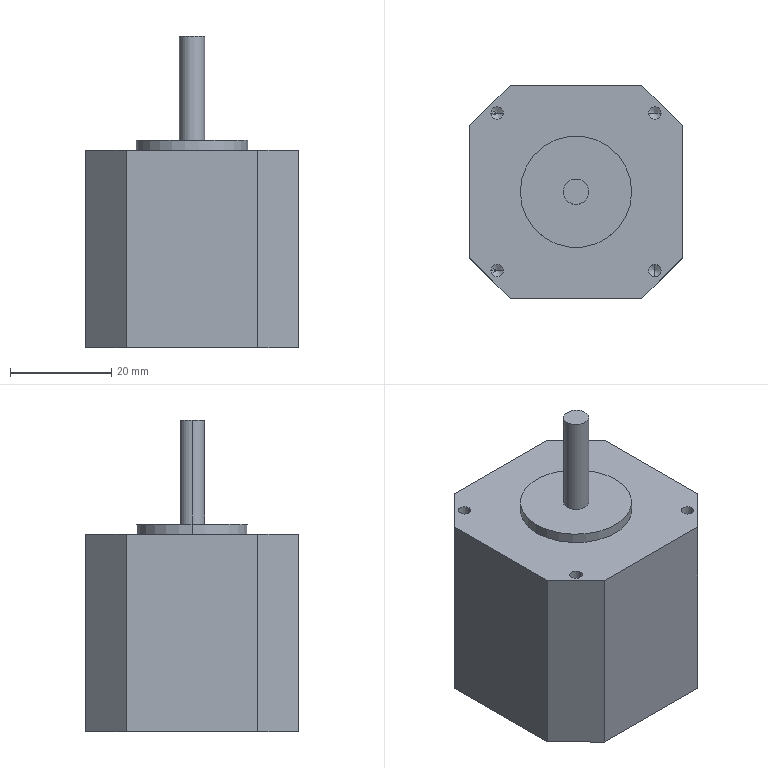Component | SolidWorks | 42StepperMotor-1 | 1 solid | 34 faces | box 42 x 42 x 61.5 mm | volume 64790 mm3 | cylinder 13 | plane 13 | cone 8 | commonest cylinder face diameters 2.5 x8 5 x3 22 x2
STEP:
#1=COLOUR_RGB('',0.7922,0.8196,0.9333);
#2=FILL_AREA_STYLE_COLOUR('',#1);
#3=FILL_AREA_STYLE('',(#2));
#4=SURFACE_STYLE_FILL_AREA(#3);
#5=SURFACE_SIDE_STYLE('',(#4));
#6=SURFACE_STYLE_USAGE(.BOTH.,#5);
#7=PRESENTATION_STYLE_ASSIGNMENT((#6));
#8=CARTESIAN_POINT('',(-0.4331,0.,0.07874));
#9=VERTEX_POINT('',#8);
#10=CARTESIAN_POINT('',(0.4331,0.,0.07874));
#11=VERTEX_POINT('',#10);
#12=CARTESIAN_POINT('',(-0.,0.,0.07874));
#13=DIRECTION('',(0.,0.,-1.));
#14=DIRECTION('',(-1.,0.,0.));
#15=AXIS2_PLACEMENT_3D('',#12,#13,#14);
#16=CIRCLE('',#15,0.4331);
#17=EDGE_CURVE('',#9,#11,#16,.T.);
#18=ORIENTED_EDGE('',*,*,#17,.T.);
#19=CARTESIAN_POINT('',(0.4331,0.,0.));
#20=VERTEX_POINT('',#19);
#21=CARTESIAN_POINT('',(0.4331,0.,0.07874));
#22=DIRECTION('',(0.,0.,-1.));
#23=VECTOR('',#22,39.37);
#24=LINE('',#21,#23);
#25=EDGE_CURVE('',#11,#20,#24,.T.);
#26=ORIENTED_EDGE('',*,*,#25,.T.);
#27=CARTESIAN_POINT('',(-0.4331,0.,0.));
#28=VERTEX_POINT('',#27);
#29=CARTESIAN_POINT('',(-0.,0.,0.));
#30=DIRECTION('',(0.,0.,1.));
#31=DIRECTION('',(-1.,0.,0.));
#32=AXIS2_PLACEMENT_3D('',#29,#30,#31);
#33=CIRCLE('',#32,0.4331);
#34=EDGE_CURVE('',#20,#28,#33,.T.);
#35=ORIENTED_EDGE('',*,*,#34,.T.);
#36=CARTESIAN_POINT('',(-0.4331,0.,0.07874));
#37=DIRECTION('',(0.,0.,-1.));
#38=VECTOR('',#37,39.37);
#39=LINE('',#36,#38);
#40=EDGE_CURVE('',#9,#28,#39,.T.);
#41=ORIENTED_EDGE('',*,*,#40,.F.);
#42=EDGE_LOOP('',(#18,#26,#35,#41));
#43=FACE_OUTER_BOUND('',#42,.T.);
#44=CARTESIAN_POINT('',(-0.,0.,0.07874));
#45=DIRECTION('',(0.,0.,-1.));
#46=DIRECTION('',(-1.,0.,0.));
#47=AXIS2_PLACEMENT_3D('',#44,#45,#46);
#48=CYLINDRICAL_SURFACE('',#47,0.4331);
#49=ADVANCED_FACE('',(#43),#48,.T.);
#50=CARTESIAN_POINT('',(-0.6617,0.6125,-0.3346));
#51=VERTEX_POINT('',#50);
#52=CARTESIAN_POINT('',(-0.5632,0.6125,-0.3346));
#53=VERTEX_POINT('',#52);
#54=CARTESIAN_POINT('',(-0.6125,0.6125,-0.3346));
#55=DIRECTION('',(0.,0.,1.));
#56=DIRECTION('',(1.,0.,0.));
#57=AXIS2_PLACEMENT_3D('',#54,#55,#56);
#58=CIRCLE('',#57,0.04921);
#59=EDGE_CURVE('',#51,#53,#58,.T.);
#60=ORIENTED_EDGE('',*,*,#59,.F.);
#61=CARTESIAN_POINT('',(-0.6617,0.6125,0.));
#62=VERTEX_POINT('',#61);
#63=CARTESIAN_POINT('',(-0.6617,0.6125,0.));
#64=DIRECTION('',(0.,0.,1.));
#65=VECTOR('',#64,39.37);
#66=LINE('',#63,#65);
#67=EDGE_CURVE('',#51,#62,#66,.T.);
#68=ORIENTED_EDGE('',*,*,#67,.T.);
#69=CARTESIAN_POINT('',(-0.5632,0.6125,0.));
#70=VERTEX_POINT('',#69);
#71=CARTESIAN_POINT('',(-0.6125,0.6125,0.));
#72=DIRECTION('',(0.,0.,1.));
#73=DIRECTION('',(1.,0.,0.));
#74=AXIS2_PLACEMENT_3D('',#71,#72,#73);
#75=CIRCLE('',#74,0.04921);
#76=EDGE_CURVE('',#62,#70,#75,.T.);
#77=ORIENTED_EDGE('',*,*,#76,.T.);
#78=CARTESIAN_POINT('',(-0.5632,0.6125,0.));
#79=DIRECTION('',(0.,0.,1.));
#80=VECTOR('',#79,39.37);
#81=LINE('',#78,#80);
#82=EDGE_CURVE('',#53,#70,#81,.T.);
#83=ORIENTED_EDGE('',*,*,#82,.F.);
#84=EDGE_LOOP('',(#60,#68,#77,#83));
#85=FACE_OUTER_BOUND('',#84,.T.);
#86=CARTESIAN_POINT('',(-0.6125,0.6125,0.));
#87=DIRECTION('',(0.,0.,1.));
#88=DIRECTION('',(1.,0.,0.));
#89=AXIS2_PLACEMENT_3D('',#86,#87,#88);
#90=CYLINDRICAL_SURFACE('',#89,0.04921);
#91=ADVANCED_FACE('',(#85),#90,.F.);
#92=CARTESIAN_POINT('',(0.5632,0.6125,-0.3346));
#93=VERTEX_POINT('',#92);
#94=CARTESIAN_POINT('',(0.6617,0.6125,-0.3346));
#95=VERTEX_POINT('',#94);
#96=CARTESIAN_POINT('',(0.6125,0.6125,-0.3346));
#97=DIRECTION('',(0.,0.,1.));
#98=DIRECTION('',(1.,0.,0.));
#99=AXIS2_PLACEMENT_3D('',#96,#97,#98);
#100=CIRCLE('',#99,0.04921);
#101=EDGE_CURVE('',#93,#95,#100,.T.);
#102=ORIENTED_EDGE('',*,*,#101,.F.);
#103=CARTESIAN_POINT('',(0.5632,0.6125,0.));
#104=VERTEX_POINT('',#103);
#105=CARTESIAN_POINT('',(0.5632,0.6125,0.));
#106=DIRECTION('',(0.,0.,1.));
#107=VECTOR('',#106,39.37);
#108=LINE('',#105,#107);
#109=EDGE_CURVE('',#93,#104,#108,.T.);
#110=ORIENTED_EDGE('',*,*,#109,.T.);
#111=CARTESIAN_POINT('',(0.6617,0.6125,0.));
#112=VERTEX_POINT('',#111);
#113=CARTESIAN_POINT('',(0.6125,0.6125,0.));
#114=DIRECTION('',(0.,0.,1.));
#115=DIRECTION('',(1.,0.,0.));
#116=AXIS2_PLACEMENT_3D('',#113,#114,#115);
#117=CIRCLE('',#116,0.04921);
#118=EDGE_CURVE('',#104,#112,#117,.T.);
#119=ORIENTED_EDGE('',*,*,#118,.T.);
#120=CARTESIAN_POINT('',(0.6617,0.6125,0.));
#121=DIRECTION('',(0.,0.,1.));
#122=VECTOR('',#121,39.37);
#123=LINE('',#120,#122);
#124=EDGE_CURVE('',#95,#112,#123,.T.);
#125=ORIENTED_EDGE('',*,*,#124,.F.);
#126=EDGE_LOOP('',(#102,#110,#119,#125));
#127=FACE_OUTER_BOUND('',#126,.T.);
#128=CARTESIAN_POINT('',(0.6125,0.6125,0.));
#129=DIRECTION('',(0.,0.,1.));
#130=DIRECTION('',(1.,0.,0.));
#131=AXIS2_PLACEMENT_3D('',#128,#129,#130);
#132=CYLINDRICAL_SURFACE('',#131,0.04921);
#133=ADVANCED_FACE('',(#127),#132,.F.);
#134=CARTESIAN_POINT('',(0.5632,-0.6125,-0.3346));
#135=VERTEX_POINT('',#134);
#136=CARTESIAN_POINT('',(0.6125,-0.6617,-0.3346));
#137=VERTEX_POINT('',#136);
#138=CARTESIAN_POINT('',(0.6125,-0.6125,-0.3346));
#139=DIRECTION('',(0.,0.,1.));
#140=DIRECTION('',(1.,0.,0.));
#141=AXIS2_PLACEMENT_3D('',#138,#139,#140);
#142=CIRCLE('',#141,0.04921);
#143=EDGE_CURVE('',#135,#137,#142,.T.);
#144=ORIENTED_EDGE('',*,*,#143,.F.);
#145=CARTESIAN_POINT('',(0.5632,-0.6125,0.));
#146=VERTEX_POINT('',#145);
#147=CARTESIAN_POINT('',(0.5632,-0.6125,0.));
#148=DIRECTION('',(0.,0.,1.));
#149=VECTOR('',#148,39.37);
#150=LINE('',#147,#149);
#151=EDGE_CURVE('',#135,#146,#150,.T.);
#152=ORIENTED_EDGE('',*,*,#151,.T.);
#153=CARTESIAN_POINT('',(0.6617,-0.6125,0.));
#154=VERTEX_POINT('',#153);
#155=CARTESIAN_POINT('',(0.6125,-0.6125,0.));
#156=DIRECTION('',(0.,0.,1.));
#157=DIRECTION('',(1.,0.,0.));
#158=AXIS2_PLACEMENT_3D('',#155,#156,#157);
#159=CIRCLE('',#158,0.04921);
#160=EDGE_CURVE('',#146,#154,#159,.T.);
#161=ORIENTED_EDGE('',*,*,#160,.T.);
#162=CARTESIAN_POINT('',(0.6617,-0.6125,-0.3346));
#163=VERTEX_POINT('',#162);
#164=CARTESIAN_POINT('',(0.6617,-0.6125,0.));
#165=DIRECTION('',(0.,0.,1.));
#166=VECTOR('',#165,39.37);
#167=LINE('',#164,#166);
#168=EDGE_CURVE('',#163,#154,#167,.T.);
#169=ORIENTED_EDGE('',*,*,#168,.F.);
#170=CARTESIAN_POINT('',(0.6125,-0.6125,-0.3346));
#171=DIRECTION('',(0.,0.,1.));
#172=DIRECTION('',(1.,0.,0.));
#173=AXIS2_PLACEMENT_3D('',#170,#171,#172);
#174=CIRCLE('',#173,0.04921);
#175=EDGE_CURVE('',#137,#163,#174,.T.);
#176=ORIENTED_EDGE('',*,*,#175,.F.);
#177=EDGE_LOOP('',(#144,#152,#161,#169,#176));
#178=FACE_OUTER_BOUND('',#177,.T.);
#179=CARTESIAN_POINT('',(0.6125,-0.6125,0.));
#180=DIRECTION('',(0.,0.,1.));
#181=DIRECTION('',(1.,0.,0.));
#182=AXIS2_PLACEMENT_3D('',#179,#180,#181);
#183=CYLINDRICAL_SURFACE('',#182,0.04921);
#184=ADVANCED_FACE('',(#178),#183,.F.);
#185=CARTESIAN_POINT('',(-0.6617,-0.6125,-0.3346));
#186=VERTEX_POINT('',#185);
#187=CARTESIAN_POINT('',(-0.5632,-0.6125,-0.3346));
#188=VERTEX_POINT('',#187);
#189=CARTESIAN_POINT('',(-0.6125,-0.6125,-0.3346));
#190=DIRECTION('',(0.,0.,1.));
#191=DIRECTION('',(1.,0.,0.));
#192=AXIS2_PLACEMENT_3D('',#189,#190,#191);
#193=CIRCLE('',#192,0.04921);
#194=EDGE_CURVE('',#186,#188,#193,.T.);
#195=ORIENTED_EDGE('',*,*,#194,.F.);
#196=CARTESIAN_POINT('',(-0.6617,-0.6125,0.));
#197=VERTEX_POINT('',#196);
#198=CARTESIAN_POINT('',(-0.6617,-0.6125,0.));
#199=DIRECTION('',(0.,0.,1.));
#200=VECTOR('',#199,39.37);
#201=LINE('',#198,#200);
#202=EDGE_CURVE('',#186,#197,#201,.T.);
#203=ORIENTED_EDGE('',*,*,#202,.T.);
#204=CARTESIAN_POINT('',(-0.5632,-0.6125,0.));
#205=VERTEX_POINT('',#204);
#206=CARTESIAN_POINT('',(-0.6125,-0.6125,0.));
#207=DIRECTION('',(0.,0.,1.));
#208=DIRECTION('',(1.,0.,0.));
#209=AXIS2_PLACEMENT_3D('',#206,#207,#208);
#210=CIRCLE('',#209,0.04921);
#211=EDGE_CURVE('',#197,#205,#210,.T.);
#212=ORIENTED_EDGE('',*,*,#211,.T.);
#213=CARTESIAN_POINT('',(-0.5632,-0.6125,0.));
#214=DIRECTION('',(0.,0.,1.));
#215=VECTOR('',#214,39.37);
#216=LINE('',#213,#215);
#217=EDGE_CURVE('',#188,#205,#216,.T.);
#218=ORIENTED_EDGE('',*,*,#217,.F.);
#219=EDGE_LOOP('',(#195,#203,#212,#218));
#220=FACE_OUTER_BOUND('',#219,.T.);
#221=CARTESIAN_POINT('',(-0.6125,-0.6125,0.));
#222=DIRECTION('',(0.,0.,1.));
#223=DIRECTION('',(1.,0.,0.));
#224=AXIS2_PLACEMENT_3D('',#221,#222,#223);
#225=CYLINDRICAL_SURFACE('',#224,0.04921);
#226=ADVANCED_FACE('',(#220),#225,.F.);
#227=CARTESIAN_POINT('',(-0.6125,0.6125,-0.3642));
#228=VERTEX_POINT('',#227);
#229=CARTESIAN_POINT('',(-0.5632,0.6125,-0.3346));
#230=DIRECTION('',(0.8572,0.,0.515));
#231=VECTOR('',#230,39.37);
#232=LINE('',#229,#231);
#233=EDGE_CURVE('',#228,#53,#232,.T.);
#234=ORIENTED_EDGE('',*,*,#233,.F.);
#235=CARTESIAN_POINT('',(-0.6617,0.6125,-0.3346));
#236=DIRECTION('',(-0.8572,0.,0.515));
#237=VECTOR('',#236,39.37);
#238=LINE('',#235,#237);
#239=EDGE_CURVE('',#228,#51,#238,.T.);
#240=ORIENTED_EDGE('',*,*,#239,.T.);
#241=ORIENTED_EDGE('',*,*,#59,.T.);
#242=EDGE_LOOP('',(#234,#240,#241));
#243=FACE_OUTER_BOUND('',#242,.T.);
#244=CARTESIAN_POINT('',(-0.6125,0.6125,-0.3346));
#245=DIRECTION('',(0.,0.,1.));
#246=DIRECTION('',(1.,0.,0.));
#247=AXIS2_PLACEMENT_3D('',#244,#245,#246);
#248=CONICAL_SURFACE('',#247,0.04921,1.03);
#249=ADVANCED_FACE('',(#243),#248,.F.);
#250=CARTESIAN_POINT('',(0.6125,0.6125,-0.3642));
#251=VERTEX_POINT('',#250);
#252=CARTESIAN_POINT('',(0.6617,0.6125,-0.3346));
#253=DIRECTION('',(0.8572,0.,0.515));
#254=VECTOR('',#253,39.37);
#255=LINE('',#252,#254);
#256=EDGE_CURVE('',#251,#95,#255,.T.);
#257=ORIENTED_EDGE('',*,*,#256,.F.);
#258=CARTESIAN_POINT('',(0.5632,0.6125,-0.3346));
#259=DIRECTION('',(-0.8572,0.,0.515));
#260=VECTOR('',#259,39.37);
#261=LINE('',#258,#260);
#262=EDGE_CURVE('',#251,#93,#261,.T.);
#263=ORIENTED_EDGE('',*,*,#262,.T.);
#264=ORIENTED_EDGE('',*,*,#101,.T.);
#265=EDGE_LOOP('',(#257,#263,#264));
#266=FACE_OUTER_BOUND('',#265,.T.);
#267=CARTESIAN_POINT('',(0.6125,0.6125,-0.3346));
#268=DIRECTION('',(0.,0.,1.));
#269=DIRECTION('',(1.,0.,0.));
#270=AXIS2_PLACEMENT_3D('',#267,#268,#269);
#271=CONICAL_SURFACE('',#270,0.04921,1.03);
#272=ADVANCED_FACE('',(#266),#271,.F.);
#273=CARTESIAN_POINT('',(0.6125,-0.6125,-0.3642));
#274=VERTEX_POINT('',#273);
#275=CARTESIAN_POINT('',(0.6125,-0.6617,-0.3346));
#276=DIRECTION('',(0.,-0.8572,0.515));
#277=VECTOR('',#276,39.37);
#278=LINE('',#275,#277);
#279=EDGE_CURVE('',#274,#137,#278,.T.);
#280=ORIENTED_EDGE('',*,*,#279,.F.);
#281=CARTESIAN_POINT('',(0.6125,-0.5632,-0.3346));
#282=VERTEX_POINT('',#281);
#283=CARTESIAN_POINT('',(0.6125,-0.5632,-0.3346));
#284=DIRECTION('',(0.,0.8572,0.515));
#285=VECTOR('',#284,39.37);
#286=LINE('',#283,#285);
#287=EDGE_CURVE('',#274,#282,#286,.T.);
#288=ORIENTED_EDGE('',*,*,#287,.T.);
#289=CARTESIAN_POINT('',(0.6125,-0.6125,-0.3346));
#290=DIRECTION('',(0.,0.,1.));
#291=DIRECTION('',(1.,0.,0.));
#292=AXIS2_PLACEMENT_3D('',#289,#290,#291);
#293=CIRCLE('',#292,0.04921);
#294=EDGE_CURVE('',#282,#135,#293,.T.);
#295=ORIENTED_EDGE('',*,*,#294,.T.);
#296=ORIENTED_EDGE('',*,*,#143,.T.);
#297=EDGE_LOOP('',(#280,#288,#295,#296));
#298=FACE_OUTER_BOUND('',#297,.T.);
#299=CARTESIAN_POINT('',(0.6125,-0.6125,-0.3346));
#300=DIRECTION('',(0.,0.,1.));
#301=DIRECTION('',(0.,-1.,0.));
#302=AXIS2_PLACEMENT_3D('',#299,#300,#301);
#303=CONICAL_SURFACE('',#302,0.04921,1.03);
#304=ADVANCED_FACE('',(#298),#303,.F.);
#305=CARTESIAN_POINT('',(-0.6125,-0.6125,-0.3642));
#306=VERTEX_POINT('',#305);
#307=CARTESIAN_POINT('',(-0.5632,-0.6125,-0.3346));
#308=DIRECTION('',(0.8572,0.,0.515));
#309=VECTOR('',#308,39.37);
#310=LINE('',#307,#309);
#311=EDGE_CURVE('',#306,#188,#310,.T.);
#312=ORIENTED_EDGE('',*,*,#311,.F.);
#313=CARTESIAN_POINT('',(-0.6617,-0.6125,-0.3346));
#314=DIRECTION('',(-0.8572,0.,0.515));
#315=VECTOR('',#314,39.37);
#316=LINE('',#313,#315);
#317=EDGE_CURVE('',#306,#186,#316,.T.);
#318=ORIENTED_EDGE('',*,*,#317,.T.);
#319=ORIENTED_EDGE('',*,*,#194,.T.);
#320=EDGE_LOOP('',(#312,#318,#319));
#321=FACE_OUTER_BOUND('',#320,.T.);
#322=CARTESIAN_POINT('',(-0.6125,-0.6125,-0.3346));
#323=DIRECTION('',(0.,0.,1.));
#324=DIRECTION('',(1.,0.,0.));
#325=AXIS2_PLACEMENT_3D('',#322,#323,#324);
#326=CONICAL_SURFACE('',#325,0.04921,1.03);
#327=ADVANCED_FACE('',(#321),#326,.F.);
#328=CARTESIAN_POINT('',(0.03857,0.09055,0.8858));
#329=VERTEX_POINT('',#328);
#330=CARTESIAN_POINT('',(0.09843,0.,0.8858));
#331=VERTEX_POINT('',#330);
#332=CARTESIAN_POINT('',(-0.,0.,0.8858));
#333=DIRECTION('',(0.,0.,-1.));
#334=DIRECTION('',(-1.,0.,0.));
#335=AXIS2_PLACEMENT_3D('',#332,#333,#334);
#336=CIRCLE('',#335,0.09843);
#337=EDGE_CURVE('',#329,#331,#336,.T.);
#338=ORIENTED_EDGE('',*,*,#337,.T.);
#339=CARTESIAN_POINT('',(0.09843,0.,0.07874));
#340=VERTEX_POINT('',#339);
#341=CARTESIAN_POINT('',(0.09843,0.,0.8858));
#342=DIRECTION('',(0.,0.,-1.));
#343=VECTOR('',#342,39.37);
#344=LINE('',#341,#343);
#345=EDGE_CURVE('',#331,#340,#344,.T.);
#346=ORIENTED_EDGE('',*,*,#345,.T.);
#347=CARTESIAN_POINT('',(0.03857,0.09055,0.07874));
#348=VERTEX_POINT('',#347);
#349=CARTESIAN_POINT('',(-0.,0.,0.07874));
#350=DIRECTION('',(0.,0.,-1.));
#351=DIRECTION('',(-1.,0.,0.));
#352=AXIS2_PLACEMENT_3D('',#349,#350,#351);
#353=CIRCLE('',#352,0.09843);
#354=EDGE_CURVE('',#348,#340,#353,.T.);
#355=ORIENTED_EDGE('',*,*,#354,.F.);
#356=CARTESIAN_POINT('',(0.03857,0.09055,0.8858));
#357=DIRECTION('',(0.,0.,1.));
#358=VECTOR('',#357,39.37);
#359=LINE('',#356,#358);
#360=EDGE_CURVE('',#348,#329,#359,.T.);
#361=ORIENTED_EDGE('',*,*,#360,.T.);
#362=EDGE_LOOP('',(#338,#346,#355,#361));
#363=FACE_OUTER_BOUND('',#362,.T.);
#364=CARTESIAN_POINT('',(-0.,0.,0.8858));
#365=DIRECTION('',(0.,0.,-1.));
#366=DIRECTION('',(-1.,0.,0.));
#367=AXIS2_PLACEMENT_3D('',#364,#365,#366);
#368=CYLINDRICAL_SURFACE('',#367,0.09843);
#369=ADVANCED_FACE('',(#363),#368,.T.);
#370=ORIENTED_EDGE('',*,*,#345,.F.);
#371=CARTESIAN_POINT('',(-0.09843,0.,0.8858));
#372=VERTEX_POINT('',#371);
#373=CARTESIAN_POINT('',(-0.,0.,0.8858));
#374=DIRECTION('',(0.,0.,-1.));
#375=DIRECTION('',(-1.,0.,0.));
#376=AXIS2_PLACEMENT_3D('',#373,#374,#375);
#377=CIRCLE('',#376,0.09843);
#378=EDGE_CURVE('',#331,#372,#377,.T.);
#379=ORIENTED_EDGE('',*,*,#378,.T.);
#380=CARTESIAN_POINT('',(-0.09843,0.,0.07874));
#381=VERTEX_POINT('',#380);
#382=CARTESIAN_POINT('',(-0.09843,0.,0.8858));
#383=DIRECTION('',(0.,0.,-1.));
#384=VECTOR('',#383,39.37);
#385=LINE('',#382,#384);
#386=EDGE_CURVE('',#372,#381,#385,.T.);
#387=ORIENTED_EDGE('',*,*,#386,.T.);
#388=CARTESIAN_POINT('',(-0.,0.,0.07874));
#389=DIRECTION('',(0.,0.,-1.));
#390=DIRECTION('',(-1.,0.,0.));
#391=AXIS2_PLACEMENT_3D('',#388,#389,#390);
#392=CIRCLE('',#391,0.09843);
#393=EDGE_CURVE('',#340,#381,#392,.T.);
#394=ORIENTED_EDGE('',*,*,#393,.F.);
#395=EDGE_LOOP('',(#370,#379,#387,#394));
#396=FACE_OUTER_BOUND('',#395,.T.);
#397=CARTESIAN_POINT('',(-0.,0.,0.8858));
#398=DIRECTION('',(0.,0.,-1.));
#399=DIRECTION('',(-1.,0.,0.));
#400=AXIS2_PLACEMENT_3D('',#397,#398,#399);
#401=CYLINDRICAL_SURFACE('',#400,0.09843);
#402=ADVANCED_FACE('',(#396),#401,.T.);
#403=CARTESIAN_POINT('',(-0.5118,0.8268,-1.535));
#404=VERTEX_POINT('',#403);
#405=CARTESIAN_POINT('',(0.5118,0.8268,-1.535));
#406=VERTEX_POINT('',#405);
#407=CARTESIAN_POINT('',(-0.,0.8268,-1.535));
#408=DIRECTION('',(1.,0.,0.));
#409=VECTOR('',#408,39.37);
#410=LINE('',#407,#409);
#411=EDGE_CURVE('',#404,#406,#410,.T.);
#412=ORIENTED_EDGE('',*,*,#411,.T.);
#413=CARTESIAN_POINT('',(0.8268,0.5118,-1.535));
#414=VERTEX_POINT('',#413);
#415=CARTESIAN_POINT('',(0.5118,0.8268,-1.535));
#416=DIRECTION('',(0.7071,-0.7071,0.));
#417=VECTOR('',#416,39.37);
#418=LINE('',#415,#417);
#419=EDGE_CURVE('',#406,#414,#418,.T.);
#420=ORIENTED_EDGE('',*,*,#419,.T.);
#421=CARTESIAN_POINT('',(0.8268,-0.5118,-1.535));
#422=VERTEX_POINT('',#421);
#423=CARTESIAN_POINT('',(0.8268,0.,-1.535));
#424=DIRECTION('',(0.,-1.,0.));
#425=VECTOR('',#424,39.37);
#426=LINE('',#423,#425);
#427=EDGE_CURVE('',#414,#422,#426,.T.);
#428=ORIENTED_EDGE('',*,*,#427,.T.);
#429=CARTESIAN_POINT('',(0.5118,-0.8268,-1.535));
#430=VERTEX_POINT('',#429);
#431=CARTESIAN_POINT('',(0.8268,-0.5118,-1.535));
#432=DIRECTION('',(-0.7071,-0.7071,0.));
#433=VECTOR('',#432,39.37);
#434=LINE('',#431,#433);
#435=EDGE_CURVE('',#422,#430,#434,.T.);
#436=ORIENTED_EDGE('',*,*,#435,.T.);
#437=CARTESIAN_POINT('',(-0.5118,-0.8268,-1.535));
#438=VERTEX_POINT('',#437);
#439=CARTESIAN_POINT('',(-0.,-0.8268,-1.535));
#440=DIRECTION('',(-1.,0.,0.));
#441=VECTOR('',#440,39.37);
#442=LINE('',#439,#441);
#443=EDGE_CURVE('',#430,#438,#442,.T.);
#444=ORIENTED_EDGE('',*,*,#443,.T.);
#445=CARTESIAN_POINT('',(-0.8268,-0.5118,-1.535));
#446=VERTEX_POINT('',#445);
#447=CARTESIAN_POINT('',(-0.5118,-0.8268,-1.535));
#448=DIRECTION('',(-0.7071,0.7071,0.));
#449=VECTOR('',#448,39.37);
#450=LINE('',#447,#449);
#451=EDGE_CURVE('',#438,#446,#450,.T.);
#452=ORIENTED_EDGE('',*,*,#451,.T.);
#453=CARTESIAN_POINT('',(-0.8268,0.5118,-1.535));
#454=VERTEX_POINT('',#453);
#455=CARTESIAN_POINT('',(-0.8268,0.,-1.535));
#456=DIRECTION('',(0.,1.,0.));
#457=VECTOR('',#456,39.37);
#458=LINE('',#455,#457);
#459=EDGE_CURVE('',#446,#454,#458,.T.);
#460=ORIENTED_EDGE('',*,*,#459,.T.);
#461=CARTESIAN_POINT('',(-0.8268,0.5118,-1.535));
#462=DIRECTION('',(0.7071,0.7071,0.));
#463=VECTOR('',#462,39.37);
#464=LINE('',#461,#463);
#465=EDGE_CURVE('',#454,#404,#464,.T.);
#466=ORIENTED_EDGE('',*,*,#465,.T.);
#467=EDGE_LOOP('',(#412,#420,#428,#436,#444,#452,#460,#466));
#468=FACE_OUTER_BOUND('',#467,.T.);
#469=CARTESIAN_POINT('',(-0.,0.,-1.535));
#470=DIRECTION('',(0.,0.,-1.));
#471=DIRECTION('',(-1.,0.,0.));
#472=AXIS2_PLACEMENT_3D('',#469,#470,#471);
#473=PLANE('',#472);
#474=ADVANCED_FACE('',(#468),#473,.T.);
#475=CARTESIAN_POINT('',(0.8268,0.5118,0.));
#476=VERTEX_POINT('',#475);
#477=CARTESIAN_POINT('',(0.8268,0.5118,0.));
#478=DIRECTION('',(0.,0.,1.));
#479=VECTOR('',#478,39.37);
#480=LINE('',#477,#479);
#481=EDGE_CURVE('',#414,#476,#480,.T.);
#482=ORIENTED_EDGE('',*,*,#481,.F.);
#483=ORIENTED_EDGE('',*,*,#419,.F.);
#484=CARTESIAN_POINT('',(0.5118,0.8268,0.));
#485=VERTEX_POINT('',#484);
#486=CARTESIAN_POINT('',(0.5118,0.8268,0.));
#487=DIRECTION('',(0.,0.,-1.));
#488=VECTOR('',#487,39.37);
#489=LINE('',#486,#488);
#490=EDGE_CURVE('',#485,#406,#489,.T.);
#491=ORIENTED_EDGE('',*,*,#490,.F.);
#492=CARTESIAN_POINT('',(0.5118,0.8268,0.));
#493=DIRECTION('',(-0.7071,0.7071,0.));
#494=VECTOR('',#493,39.37);
#495=LINE('',#492,#494);
#496=EDGE_CURVE('',#476,#485,#495,.T.);
#497=ORIENTED_EDGE('',*,*,#496,.F.);
#498=EDGE_LOOP('',(#482,#483,#491,#497));
#499=FACE_OUTER_BOUND('',#498,.T.);
#500=CARTESIAN_POINT('',(0.5118,0.8268,0.));
#501=DIRECTION('',(-0.7071,-0.7071,0.));
#502=DIRECTION('',(0.7071,-0.7071,0.));
#503=AXIS2_PLACEMENT_3D('',#500,#501,#502);
#504=PLANE('',#503);
#505=ADVANCED_FACE('',(#499),#504,.F.);
#506=CARTESIAN_POINT('',(-0.5118,0.8268,0.));
#507=VERTEX_POINT('',#506);
#508=CARTESIAN_POINT('',(-0.5118,0.8268,0.));
#509=DIRECTION('',(0.,0.,-1.));
#510=VECTOR('',#509,39.37);
#511=LINE('',#508,#510);
#512=EDGE_CURVE('',#507,#404,#511,.T.);
#513=ORIENTED_EDGE('',*,*,#512,.F.);
#514=CARTESIAN_POINT('',(-0.8268,0.8268,0.));
#515=DIRECTION('',(-1.,0.,0.));
#516=VECTOR('',#515,39.37);
#517=LINE('',#514,#516);
#518=EDGE_CURVE('',#485,#507,#517,.T.);
#519=ORIENTED_EDGE('',*,*,#518,.F.);
#520=ORIENTED_EDGE('',*,*,#490,.T.);
#521=ORIENTED_EDGE('',*,*,#411,.F.);
#522=EDGE_LOOP('',(#513,#519,#520,#521));
#523=FACE_OUTER_BOUND('',#522,.T.);
#524=CARTESIAN_POINT('',(-0.8268,0.8268,0.));
#525=DIRECTION('',(0.,-1.,0.));
#526=DIRECTION('',(0.,0.,-1.));
#527=AXIS2_PLACEMENT_3D('',#524,#525,#526);
#528=PLANE('',#527);
#529=ADVANCED_FACE('',(#523),#528,.F.);
#530=ORIENTED_EDGE('',*,*,#512,.T.);
#531=ORIENTED_EDGE('',*,*,#465,.F.);
#532=CARTESIAN_POINT('',(-0.8268,0.5118,0.));
#533=VERTEX_POINT('',#532);
#534=CARTESIAN_POINT('',(-0.8268,0.5118,0.));
#535=DIRECTION('',(0.,0.,-1.));
#536=VECTOR('',#535,39.37);
#537=LINE('',#534,#536);
#538=EDGE_CURVE('',#533,#454,#537,.T.);
#539=ORIENTED_EDGE('',*,*,#538,.F.);
#540=CARTESIAN_POINT('',(-0.8268,0.5118,0.));
#541=DIRECTION('',(-0.7071,-0.7071,0.));
#542=VECTOR('',#541,39.37);
#543=LINE('',#540,#542);
#544=EDGE_CURVE('',#507,#533,#543,.T.);
#545=ORIENTED_EDGE('',*,*,#544,.F.);
#546=EDGE_LOOP('',(#530,#531,#539,#545));
#547=FACE_OUTER_BOUND('',#546,.T.);
#548=CARTESIAN_POINT('',(-0.8268,0.5118,0.));
#549=DIRECTION('',(0.7071,-0.7071,0.));
#550=DIRECTION('',(0.7071,0.7071,0.));
#551=AXIS2_PLACEMENT_3D('',#548,#549,#550);
#552=PLANE('',#551);
#553=ADVANCED_FACE('',(#547),#552,.F.);
#554=CARTESIAN_POINT('',(-0.8268,-0.5118,0.));
#555=VERTEX_POINT('',#554);
#556=CARTESIAN_POINT('',(-0.8268,-0.5118,0.));
#557=DIRECTION('',(0.,0.,-1.));
#558=VECTOR('',#557,39.37);
#559=LINE('',#556,#558);
#560=EDGE_CURVE('',#555,#446,#559,.T.);
#561=ORIENTED_EDGE('',*,*,#560,.F.);
#562=CARTESIAN_POINT('',(-0.8268,-0.8268,0.));
#563=DIRECTION('',(0.,-1.,0.));
#564=VECTOR('',#563,39.37);
#565=LINE('',#562,#564);
#566=EDGE_CURVE('',#533,#555,#565,.T.);
#567=ORIENTED_EDGE('',*,*,#566,.F.);
#568=ORIENTED_EDGE('',*,*,#538,.T.);
#569=ORIENTED_EDGE('',*,*,#459,.F.);
#570=EDGE_LOOP('',(#561,#567,#568,#569));
#571=FACE_OUTER_BOUND('',#570,.T.);
#572=CARTESIAN_POINT('',(-0.8268,-0.8268,0.));
#573=DIRECTION('',(1.,0.,0.));
#574=DIRECTION('',(0.,0.,-1.));
#575=AXIS2_PLACEMENT_3D('',#572,#573,#574);
#576=PLANE('',#575);
#577=ADVANCED_FACE('',(#571),#576,.F.);
#578=ORIENTED_EDGE('',*,*,#560,.T.);
#579=ORIENTED_EDGE('',*,*,#451,.F.);
#580=CARTESIAN_POINT('',(-0.5118,-0.8268,0.));
#581=VERTEX_POINT('',#580);
#582=CARTESIAN_POINT('',(-0.5118,-0.8268,0.));
#583=DIRECTION('',(0.,0.,-1.));
#584=VECTOR('',#583,39.37);
#585=LINE('',#582,#584);
#586=EDGE_CURVE('',#581,#438,#585,.T.);
#587=ORIENTED_EDGE('',*,*,#586,.F.);
#588=CARTESIAN_POINT('',(-0.5118,-0.8268,0.));
#589=DIRECTION('',(0.7071,-0.7071,0.));
#590=VECTOR('',#589,39.37);
#591=LINE('',#588,#590);
#592=EDGE_CURVE('',#555,#581,#591,.T.);
#593=ORIENTED_EDGE('',*,*,#592,.F.);
#594=EDGE_LOOP('',(#578,#579,#587,#593));
#595=FACE_OUTER_BOUND('',#594,.T.);
#596=CARTESIAN_POINT('',(-0.5118,-0.8268,0.));
#597=DIRECTION('',(0.7071,0.7071,0.));
#598=DIRECTION('',(-0.7071,0.7071,0.));
#599=AXIS2_PLACEMENT_3D('',#596,#597,#598);
#600=PLANE('',#599);
#601=ADVANCED_FACE('',(#595),#600,.F.);
#602=CARTESIAN_POINT('',(0.5118,-0.8268,0.));
#603=VERTEX_POINT('',#602);
#604=CARTESIAN_POINT('',(0.5118,-0.8268,0.));
#605=DIRECTION('',(0.,0.,-1.));
#606=VECTOR('',#605,39.37);
#607=LINE('',#604,#606);
#608=EDGE_CURVE('',#603,#430,#607,.T.);
#609=ORIENTED_EDGE('',*,*,#608,.F.);
#610=CARTESIAN_POINT('',(-0.8268,-0.8268,0.));
#611=DIRECTION('',(1.,0.,0.));
#612=VECTOR('',#611,39.37);
#613=LINE('',#610,#612);
#614=EDGE_CURVE('',#581,#603,#613,.T.);
#615=ORIENTED_EDGE('',*,*,#614,.F.);
#616=ORIENTED_EDGE('',*,*,#586,.T.);
#617=ORIENTED_EDGE('',*,*,#443,.F.);
#618=EDGE_LOOP('',(#609,#615,#616,#617));
#619=FACE_OUTER_BOUND('',#618,.T.);
#620=CARTESIAN_POINT('',(-0.8268,-0.8268,0.));
#621=DIRECTION('',(0.,1.,0.));
#622=DIRECTION('',(0.,0.,1.));
#623=AXIS2_PLACEMENT_3D('',#620,#621,#622);
#624=PLANE('',#623);
#625=ADVANCED_FACE('',(#619),#624,.F.);
#626=ORIENTED_EDGE('',*,*,#608,.T.);
#627=ORIENTED_EDGE('',*,*,#435,.F.);
#628=CARTESIAN_POINT('',(0.8268,-0.5118,0.));
#629=VERTEX_POINT('',#628);
#630=CARTESIAN_POINT('',(0.8268,-0.5118,0.));
#631=DIRECTION('',(0.,0.,-1.));
#632=VECTOR('',#631,39.37);
#633=LINE('',#630,#632);
#634=EDGE_CURVE('',#629,#422,#633,.T.);
#635=ORIENTED_EDGE('',*,*,#634,.F.);
#636=CARTESIAN_POINT('',(0.8268,-0.5118,0.));
#637=DIRECTION('',(0.7071,0.7071,0.));
#638=VECTOR('',#637,39.37);
#639=LINE('',#636,#638);
#640=EDGE_CURVE('',#603,#629,#639,.T.);
#641=ORIENTED_EDGE('',*,*,#640,.F.);
#642=EDGE_LOOP('',(#626,#627,#635,#641));
#643=FACE_OUTER_BOUND('',#642,.T.);
#644=CARTESIAN_POINT('',(0.8268,-0.5118,0.));
#645=DIRECTION('',(-0.7071,0.7071,0.));
#646=DIRECTION('',(-0.7071,-0.7071,0.));
#647=AXIS2_PLACEMENT_3D('',#644,#645,#646);
#648=PLANE('',#647);
#649=ADVANCED_FACE('',(#643),#648,.F.);
#650=ORIENTED_EDGE('',*,*,#634,.T.);
#651=ORIENTED_EDGE('',*,*,#427,.F.);
#652=ORIENTED_EDGE('',*,*,#481,.T.);
#653=CARTESIAN_POINT('',(0.8268,-0.8268,0.));
#654=DIRECTION('',(0.,1.,0.));
#655=VECTOR('',#654,39.37);
#656=LINE('',#653,#655);
#657=EDGE_CURVE('',#629,#476,#656,.T.);
#658=ORIENTED_EDGE('',*,*,#657,.F.);
#659=EDGE_LOOP('',(#650,#651,#652,#658));
#660=FACE_OUTER_BOUND('',#659,.T.);
#661=CARTESIAN_POINT('',(0.8268,-0.8268,0.));
#662=DIRECTION('',(-1.,0.,0.));
#663=DIRECTION('',(0.,0.,1.));
#664=AXIS2_PLACEMENT_3D('',#661,#662,#663);
#665=PLANE('',#664);
#666=ADVANCED_FACE('',(#660),#665,.F.);
#667=CARTESIAN_POINT('',(-0.,0.,0.));
#668=DIRECTION('',(0.,0.,1.));
#669=DIRECTION('',(-1.,0.,0.));
#670=AXIS2_PLACEMENT_3D('',#667,#668,#669);
#671=CIRCLE('',#670,0.4331);
#672=EDGE_CURVE('',#28,#20,#671,.T.);
#673=ORIENTED_EDGE('',*,*,#672,.F.);
#674=ORIENTED_EDGE('',*,*,#34,.F.);
#675=EDGE_LOOP('',(#673,#674));
#676=FACE_BOUND('',#675,.T.);
#677=ORIENTED_EDGE('',*,*,#640,.T.);
#678=ORIENTED_EDGE('',*,*,#657,.T.);
#679=ORIENTED_EDGE('',*,*,#496,.T.);
#680=ORIENTED_EDGE('',*,*,#518,.T.);
#681=ORIENTED_EDGE('',*,*,#544,.T.);
#682=ORIENTED_EDGE('',*,*,#566,.T.);
#683=ORIENTED_EDGE('',*,*,#592,.T.);
#684=ORIENTED_EDGE('',*,*,#614,.T.);
#685=EDGE_LOOP('',(#677,#678,#679,#680,#681,#682,#683,#684));
#686=FACE_OUTER_BOUND('',#685,.T.);
#687=CARTESIAN_POINT('',(-0.6125,0.6125,0.));
#688=DIRECTION('',(0.,0.,1.));
#689=DIRECTION('',(1.,0.,0.));
#690=AXIS2_PLACEMENT_3D('',#687,#688,#689);
#691=CIRCLE('',#690,0.04921);
#692=EDGE_CURVE('',#70,#62,#691,.T.);
#693=ORIENTED_EDGE('',*,*,#692,.F.);
#694=ORIENTED_EDGE('',*,*,#76,.F.);
#695=EDGE_LOOP('',(#693,#694));
#696=FACE_BOUND('',#695,.T.);
#697=CARTESIAN_POINT('',(0.6125,0.6125,0.));
#698=DIRECTION('',(0.,0.,1.));
#699=DIRECTION('',(1.,0.,0.));
#700=AXIS2_PLACEMENT_3D('',#697,#698,#699);
#701=CIRCLE('',#700,0.04921);
#702=EDGE_CURVE('',#112,#104,#701,.T.);
#703=ORIENTED_EDGE('',*,*,#702,.F.);
#704=ORIENTED_EDGE('',*,*,#118,.F.);
#705=EDGE_LOOP('',(#703,#704));
#706=FACE_BOUND('',#705,.T.);
#707=CARTESIAN_POINT('',(0.6125,-0.6125,0.));
#708=DIRECTION('',(0.,0.,1.));
#709=DIRECTION('',(1.,0.,0.));
#710=AXIS2_PLACEMENT_3D('',#707,#708,#709);
#711=CIRCLE('',#710,0.04921);
#712=EDGE_CURVE('',#154,#146,#711,.T.);
#713=ORIENTED_EDGE('',*,*,#712,.F.);
#714=ORIENTED_EDGE('',*,*,#160,.F.);
#715=EDGE_LOOP('',(#713,#714));
#716=FACE_BOUND('',#715,.T.);
#717=CARTESIAN_POINT('',(-0.6125,-0.6125,0.));
#718=DIRECTION('',(0.,0.,1.));
#719=DIRECTION('',(1.,0.,0.));
#720=AXIS2_PLACEMENT_3D('',#717,#718,#719);
#721=CIRCLE('',#720,0.04921);
#722=EDGE_CURVE('',#205,#197,#721,.T.);
#723=ORIENTED_EDGE('',*,*,#722,.F.);
#724=ORIENTED_EDGE('',*,*,#211,.F.);
#725=EDGE_LOOP('',(#723,#724));
#726=FACE_BOUND('',#725,.T.);
#727=CARTESIAN_POINT('',(-0.,0.,0.));
#728=DIRECTION('',(0.,0.,-1.));
#729=DIRECTION('',(-1.,0.,0.));
#730=AXIS2_PLACEMENT_3D('',#727,#728,#729);
#731=PLANE('',#730);
#732=ADVANCED_FACE('',(#676,#686,#696,#706,#716,#726),#731,.F.);
#733=ORIENTED_EDGE('',*,*,#25,.F.);
#734=CARTESIAN_POINT('',(-0.,0.,0.07874));
#735=DIRECTION('',(0.,0.,-1.));
#736=DIRECTION('',(-1.,0.,0.));
#737=AXIS2_PLACEMENT_3D('',#734,#735,#736);
#738=CIRCLE('',#737,0.4331);
#739=EDGE_CURVE('',#11,#9,#738,.T.);
#740=ORIENTED_EDGE('',*,*,#739,.T.);
#741=ORIENTED_EDGE('',*,*,#40,.T.);
#742=ORIENTED_EDGE('',*,*,#672,.T.);
#743=EDGE_LOOP('',(#733,#740,#741,#742));
#744=FACE_OUTER_BOUND('',#743,.T.);
#745=CARTESIAN_POINT('',(-0.,0.,0.07874));
#746=DIRECTION('',(0.,0.,-1.));
#747=DIRECTION('',(-1.,0.,0.));
#748=AXIS2_PLACEMENT_3D('',#745,#746,#747);
#749=CYLINDRICAL_SURFACE('',#748,0.4331);
#750=ADVANCED_FACE('',(#744),#749,.T.);
#751=ORIENTED_EDGE('',*,*,#67,.F.);
#752=CARTESIAN_POINT('',(-0.6125,0.6125,-0.3346));
#753=DIRECTION('',(0.,0.,1.));
#754=DIRECTION('',(1.,0.,0.));
#755=AXIS2_PLACEMENT_3D('',#752,#753,#754);
#756=CIRCLE('',#755,0.04921);
#757=EDGE_CURVE('',#53,#51,#756,.T.);
#758=ORIENTED_EDGE('',*,*,#757,.F.);
#759=ORIENTED_EDGE('',*,*,#82,.T.);
#760=ORIENTED_EDGE('',*,*,#692,.T.);
#761=EDGE_LOOP('',(#751,#758,#759,#760));
#762=FACE_OUTER_BOUND('',#761,.T.);
#763=CARTESIAN_POINT('',(-0.6125,0.6125,0.));
#764=DIRECTION('',(0.,0.,1.));
#765=DIRECTION('',(1.,0.,0.));
#766=AXIS2_PLACEMENT_3D('',#763,#764,#765);
#767=CYLINDRICAL_SURFACE('',#766,0.04921);
#768=ADVANCED_FACE('',(#762),#767,.F.);
#769=ORIENTED_EDGE('',*,*,#109,.F.);
#770=CARTESIAN_POINT('',(0.6125,0.6125,-0.3346));
#771=DIRECTION('',(0.,0.,1.));
#772=DIRECTION('',(1.,0.,0.));
#773=AXIS2_PLACEMENT_3D('',#770,#771,#772);
#774=CIRCLE('',#773,0.04921);
#775=EDGE_CURVE('',#95,#93,#774,.T.);
#776=ORIENTED_EDGE('',*,*,#775,.F.);
#777=ORIENTED_EDGE('',*,*,#124,.T.);
#778=ORIENTED_EDGE('',*,*,#702,.T.);
#779=EDGE_LOOP('',(#769,#776,#777,#778));
#780=FACE_OUTER_BOUND('',#779,.T.);
#781=CARTESIAN_POINT('',(0.6125,0.6125,0.));
#782=DIRECTION('',(0.,0.,1.));
#783=DIRECTION('',(1.,0.,0.));
#784=AXIS2_PLACEMENT_3D('',#781,#782,#783);
#785=CYLINDRICAL_SURFACE('',#784,0.04921);
#786=ADVANCED_FACE('',(#780),#785,.F.);
#787=ORIENTED_EDGE('',*,*,#151,.F.);
#788=ORIENTED_EDGE('',*,*,#294,.F.);
#789=CARTESIAN_POINT('',(0.6125,-0.6125,-0.3346));
#790=DIRECTION('',(0.,0.,1.));
#791=DIRECTION('',(1.,0.,0.));
#792=AXIS2_PLACEMENT_3D('',#789,#790,#791);
#793=CIRCLE('',#792,0.04921);
#794=EDGE_CURVE('',#163,#282,#793,.T.);
#795=ORIENTED_EDGE('',*,*,#794,.F.);
#796=ORIENTED_EDGE('',*,*,#168,.T.);
#797=ORIENTED_EDGE('',*,*,#712,.T.);
#798=EDGE_LOOP('',(#787,#788,#795,#796,#797));
#799=FACE_OUTER_BOUND('',#798,.T.);
#800=CARTESIAN_POINT('',(0.6125,-0.6125,0.));
#801=DIRECTION('',(0.,0.,1.));
#802=DIRECTION('',(1.,0.,0.));
#803=AXIS2_PLACEMENT_3D('',#800,#801,#802);
#804=CYLINDRICAL_SURFACE('',#803,0.04921);
#805=ADVANCED_FACE('',(#799),#804,.F.);
#806=ORIENTED_EDGE('',*,*,#202,.F.);
#807=CARTESIAN_POINT('',(-0.6125,-0.6125,-0.3346));
#808=DIRECTION('',(0.,0.,1.));
#809=DIRECTION('',(1.,0.,0.));
#810=AXIS2_PLACEMENT_3D('',#807,#808,#809);
#811=CIRCLE('',#810,0.04921);
#812=EDGE_CURVE('',#188,#186,#811,.T.);
#813=ORIENTED_EDGE('',*,*,#812,.F.);
#814=ORIENTED_EDGE('',*,*,#217,.T.);
#815=ORIENTED_EDGE('',*,*,#722,.T.);
#816=EDGE_LOOP('',(#806,#813,#814,#815));
#817=FACE_OUTER_BOUND('',#816,.T.);
#818=CARTESIAN_POINT('',(-0.6125,-0.6125,0.));
#819=DIRECTION('',(0.,0.,1.));
#820=DIRECTION('',(1.,0.,0.));
#821=AXIS2_PLACEMENT_3D('',#818,#819,#820);
#822=CYLINDRICAL_SURFACE('',#821,0.04921);
#823=ADVANCED_FACE('',(#817),#822,.F.);
#824=CARTESIAN_POINT('',(-0.03857,0.09055,0.07874));
#825=VERTEX_POINT('',#824);
#826=CARTESIAN_POINT('',(-0.,0.09055,0.07874));
#827=DIRECTION('',(1.,0.,0.));
#828=VECTOR('',#827,39.37);
#829=LINE('',#826,#828);
#830=EDGE_CURVE('',#825,#348,#829,.T.);
#831=ORIENTED_EDGE('',*,*,#830,.T.);
#832=ORIENTED_EDGE('',*,*,#354,.T.);
#833=ORIENTED_EDGE('',*,*,#393,.T.);
#834=CARTESIAN_POINT('',(-0.,0.,0.07874));
#835=DIRECTION('',(0.,0.,-1.));
#836=DIRECTION('',(-1.,0.,0.));
#837=AXIS2_PLACEMENT_3D('',#834,#835,#836);
#838=CIRCLE('',#837,0.09843);
#839=EDGE_CURVE('',#381,#825,#838,.T.);
#840=ORIENTED_EDGE('',*,*,#839,.T.);
#841=EDGE_LOOP('',(#831,#832,#833,#840));
#842=FACE_BOUND('',#841,.T.);
#843=ORIENTED_EDGE('',*,*,#17,.F.);
#844=ORIENTED_EDGE('',*,*,#739,.F.);
#845=EDGE_LOOP('',(#843,#844));
#846=FACE_OUTER_BOUND('',#845,.T.);
#847=CARTESIAN_POINT('',(-0.,0.,0.07874));
#848=DIRECTION('',(0.,0.,1.));
#849=DIRECTION('',(1.,0.,0.));
#850=AXIS2_PLACEMENT_3D('',#847,#848,#849);
#851=PLANE('',#850);
#852=ADVANCED_FACE('',(#842,#846),#851,.T.);
#853=ORIENTED_EDGE('',*,*,#239,.F.);
#854=ORIENTED_EDGE('',*,*,#233,.T.);
#855=ORIENTED_EDGE('',*,*,#757,.T.);
#856=EDGE_LOOP('',(#853,#854,#855));
#857=FACE_OUTER_BOUND('',#856,.T.);
#858=CARTESIAN_POINT('',(-0.6125,0.6125,-0.3346));
#859=DIRECTION('',(0.,0.,1.));
#860=DIRECTION('',(1.,0.,0.));
#861=AXIS2_PLACEMENT_3D('',#858,#859,#860);
#862=CONICAL_SURFACE('',#861,0.04921,1.03);
#863=ADVANCED_FACE('',(#857),#862,.F.);
#864=ORIENTED_EDGE('',*,*,#262,.F.);
#865=ORIENTED_EDGE('',*,*,#256,.T.);
#866=ORIENTED_EDGE('',*,*,#775,.T.);
#867=EDGE_LOOP('',(#864,#865,#866));
#868=FACE_OUTER_BOUND('',#867,.T.);
#869=CARTESIAN_POINT('',(0.6125,0.6125,-0.3346));
#870=DIRECTION('',(0.,0.,1.));
#871=DIRECTION('',(1.,0.,0.));
#872=AXIS2_PLACEMENT_3D('',#869,#870,#871);
#873=CONICAL_SURFACE('',#872,0.04921,1.03);
#874=ADVANCED_FACE('',(#868),#873,.F.);
#875=ORIENTED_EDGE('',*,*,#287,.F.);
#876=ORIENTED_EDGE('',*,*,#279,.T.);
#877=ORIENTED_EDGE('',*,*,#175,.T.);
#878=ORIENTED_EDGE('',*,*,#794,.T.);
#879=EDGE_LOOP('',(#875,#876,#877,#878));
#880=FACE_OUTER_BOUND('',#879,.T.);
#881=CARTESIAN_POINT('',(0.6125,-0.6125,-0.3346));
#882=DIRECTION('',(0.,0.,1.));
#883=DIRECTION('',(0.,-1.,0.));
#884=AXIS2_PLACEMENT_3D('',#881,#882,#883);
#885=CONICAL_SURFACE('',#884,0.04921,1.03);
#886=ADVANCED_FACE('',(#880),#885,.F.);
#887=ORIENTED_EDGE('',*,*,#317,.F.);
#888=ORIENTED_EDGE('',*,*,#311,.T.);
#889=ORIENTED_EDGE('',*,*,#812,.T.);
#890=EDGE_LOOP('',(#887,#888,#889));
#891=FACE_OUTER_BOUND('',#890,.T.);
#892=CARTESIAN_POINT('',(-0.6125,-0.6125,-0.3346));
#893=DIRECTION('',(0.,0.,1.));
#894=DIRECTION('',(1.,0.,0.));
#895=AXIS2_PLACEMENT_3D('',#892,#893,#894);
#896=CONICAL_SURFACE('',#895,0.04921,1.03);
#897=ADVANCED_FACE('',(#891),#896,.F.);
#898=ORIENTED_EDGE('',*,*,#386,.F.);
#899=CARTESIAN_POINT('',(-0.03857,0.09055,0.8858));
#900=VERTEX_POINT('',#899);
#901=CARTESIAN_POINT('',(-0.,0.,0.8858));
#902=DIRECTION('',(0.,0.,-1.));
#903=DIRECTION('',(-1.,0.,0.));
#904=AXIS2_PLACEMENT_3D('',#901,#902,#903);
#905=CIRCLE('',#904,0.09843);
#906=EDGE_CURVE('',#372,#900,#905,.T.);
#907=ORIENTED_EDGE('',*,*,#906,.T.);
#908=CARTESIAN_POINT('',(-0.03857,0.09055,0.8858));
#909=DIRECTION('',(0.,0.,-1.));
#910=VECTOR('',#909,39.37);
#911=LINE('',#908,#910);
#912=EDGE_CURVE('',#900,#825,#911,.T.);
#913=ORIENTED_EDGE('',*,*,#912,.T.);
#914=ORIENTED_EDGE('',*,*,#839,.F.);
#915=EDGE_LOOP('',(#898,#907,#913,#914));
#916=FACE_OUTER_BOUND('',#915,.T.);
#917=CARTESIAN_POINT('',(-0.,0.,0.8858));
#918=DIRECTION('',(0.,0.,-1.));
#919=DIRECTION('',(-1.,0.,0.));
#920=AXIS2_PLACEMENT_3D('',#917,#918,#919);
#921=CYLINDRICAL_SURFACE('',#920,0.09843);
#922=ADVANCED_FACE('',(#916),#921,.T.);
#923=ORIENTED_EDGE('',*,*,#912,.F.);
#924=CARTESIAN_POINT('',(-0.03857,0.09055,0.8858));
#925=DIRECTION('',(-1.,0.,0.));
#926=VECTOR('',#925,39.37);
#927=LINE('',#924,#926);
#928=EDGE_CURVE('',#329,#900,#927,.T.);
#929=ORIENTED_EDGE('',*,*,#928,.F.);
#930=ORIENTED_EDGE('',*,*,#360,.F.);
#931=ORIENTED_EDGE('',*,*,#830,.F.);
#932=EDGE_LOOP('',(#923,#929,#930,#931));
#933=FACE_OUTER_BOUND('',#932,.T.);
#934=CARTESIAN_POINT('',(-0.03857,0.09055,0.8858));
#935=DIRECTION('',(0.,-1.,0.));
#936=DIRECTION('',(0.,0.,-1.));
#937=AXIS2_PLACEMENT_3D('',#934,#935,#936);
#938=PLANE('',#937);
#939=ADVANCED_FACE('',(#933),#938,.F.);
#940=ORIENTED_EDGE('',*,*,#337,.F.);
#941=ORIENTED_EDGE('',*,*,#928,.T.);
#942=ORIENTED_EDGE('',*,*,#906,.F.);
#943=ORIENTED_EDGE('',*,*,#378,.F.);
#944=EDGE_LOOP('',(#940,#941,#942,#943));
#945=FACE_OUTER_BOUND('',#944,.T.);
#946=CARTESIAN_POINT('',(-0.,0.,0.8858));
#947=DIRECTION('',(0.,0.,1.));
#948=DIRECTION('',(1.,0.,0.));
#949=AXIS2_PLACEMENT_3D('',#946,#947,#948);
#950=PLANE('',#949);
#951=ADVANCED_FACE('',(#945),#950,.T.);
#952=CLOSED_SHELL('',(#49,#91,#133,#184,#226,#249,#272,#304,#327,#369,#402,#474,#505,#529,#553,#577,#601,#625,#649,#666,#732,#750,#768,#786,#805,#823,#852,#863,#874,#886,#897,#922,#939,#951));
#953=MANIFOLD_SOLID_BREP('',#952);
#954=STYLED_ITEM('',(#7),#953);
#955=PRESENTATION_LAYER_ASSIGNMENT('','',(#954));
#956=CARTESIAN_POINT('',(0.,0.,0.));
#957=DIRECTION('',(0.,0.,1.));
#958=DIRECTION('',(1.,0.,0.));
#959=AXIS2_PLACEMENT_3D('',#956,#957,#958);
#960=(LENGTH_UNIT()NAMED_UNIT(*)SI_UNIT($,.METRE.));
#961=LENGTH_MEASURE_WITH_UNIT(LENGTH_MEASURE(0.0254),#960);
#962=DIMENSIONAL_EXPONENTS(1.,0.,0.,0.,0.,0.,0.);
#963=(CONVERSION_BASED_UNIT('',#961)LENGTH_UNIT()NAMED_UNIT(#962));
#964=UNCERTAINTY_MEASURE_WITH_UNIT(LENGTH_MEASURE(0.00001),#963,'','');
#965=(NAMED_UNIT(*)PLANE_ANGLE_UNIT()SI_UNIT($,.RADIAN.));
#966=(NAMED_UNIT(*)SI_UNIT($,.STERADIAN.)SOLID_ANGLE_UNIT());
#967=(GEOMETRIC_REPRESENTATION_CONTEXT(3)GLOBAL_UNCERTAINTY_ASSIGNED_CONTEXT((#964))GLOBAL_UNIT_ASSIGNED_CONTEXT((#963,#965,#966))REPRESENTATION_CONTEXT('',''));
#968=ADVANCED_BREP_SHAPE_REPRESENTATION('',(#953,#959),#967);
#969=(LENGTH_UNIT()NAMED_UNIT(*)SI_UNIT($,.METRE.));
#970=LENGTH_MEASURE_WITH_UNIT(LENGTH_MEASURE(0.0254),#969);
#971=DIMENSIONAL_EXPONENTS(1.,0.,0.,0.,0.,0.,0.);
#972=(CONVERSION_BASED_UNIT('',#970)LENGTH_UNIT()NAMED_UNIT(#971));
#973=UNCERTAINTY_MEASURE_WITH_UNIT(LENGTH_MEASURE(0.00001),#972,'','');
#974=(NAMED_UNIT(*)PLANE_ANGLE_UNIT()SI_UNIT($,.RADIAN.));
#975=(NAMED_UNIT(*)SI_UNIT($,.STERADIAN.)SOLID_ANGLE_UNIT());
#976=(GEOMETRIC_REPRESENTATION_CONTEXT(3)GLOBAL_UNCERTAINTY_ASSIGNED_CONTEXT((#973))GLOBAL_UNIT_ASSIGNED_CONTEXT((#972,#974,#975))REPRESENTATION_CONTEXT('',''));
#977=MECHANICAL_DESIGN_GEOMETRIC_PRESENTATION_REPRESENTATION('',(#954),#976);